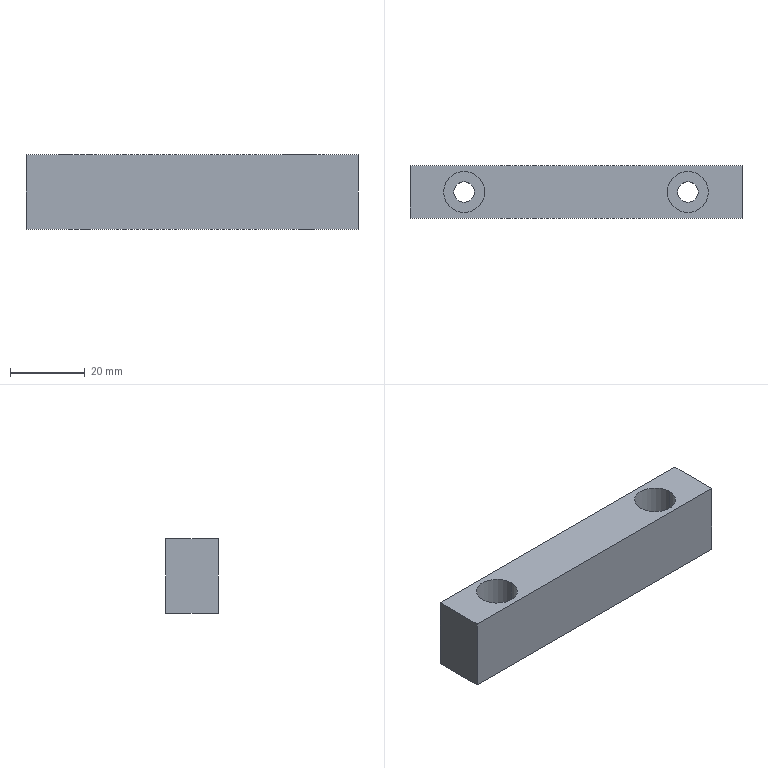CAM job | Mastercam | mm | 9 operations | part box 89 x 14 x 20
1. Facing | 20 - 63 平铣刀
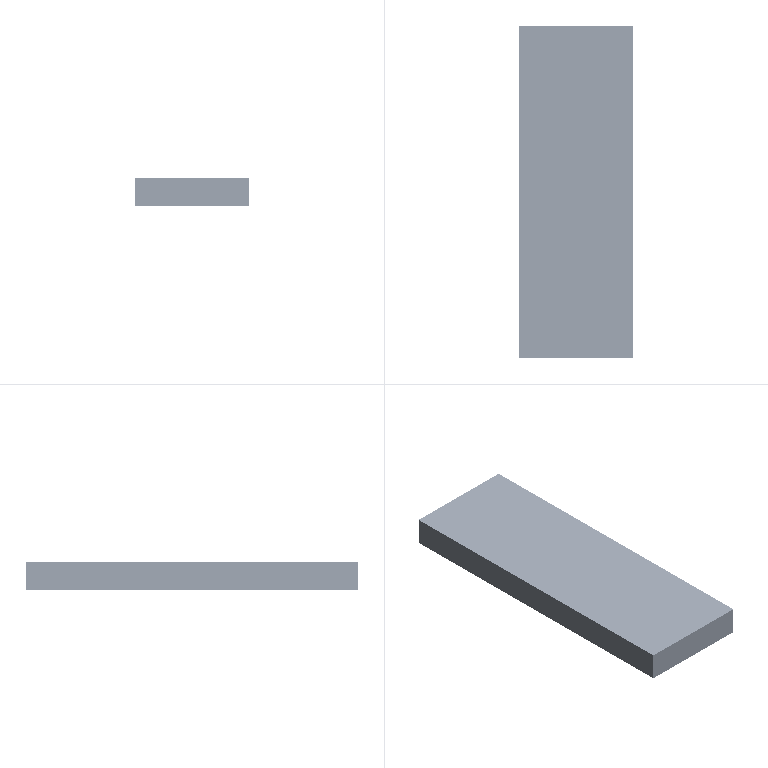2. Contour (Ramp) | 10 - 10 平铣刀
3. Contour (2D) | 10 - 10 平铣刀
4. Contour (Ramp) | 6 - 6 平铣刀
5. Contour (2D) | 6 - 6 平铣刀
6. Contour (2D chamfer) | 7 - 4 倒角刀
7. Facing | 20 - 63 平铣刀
8. Drill/Counterbore | 7 - 4 倒角刀
9. Contour (2D chamfer) | 7 - 4 倒角刀